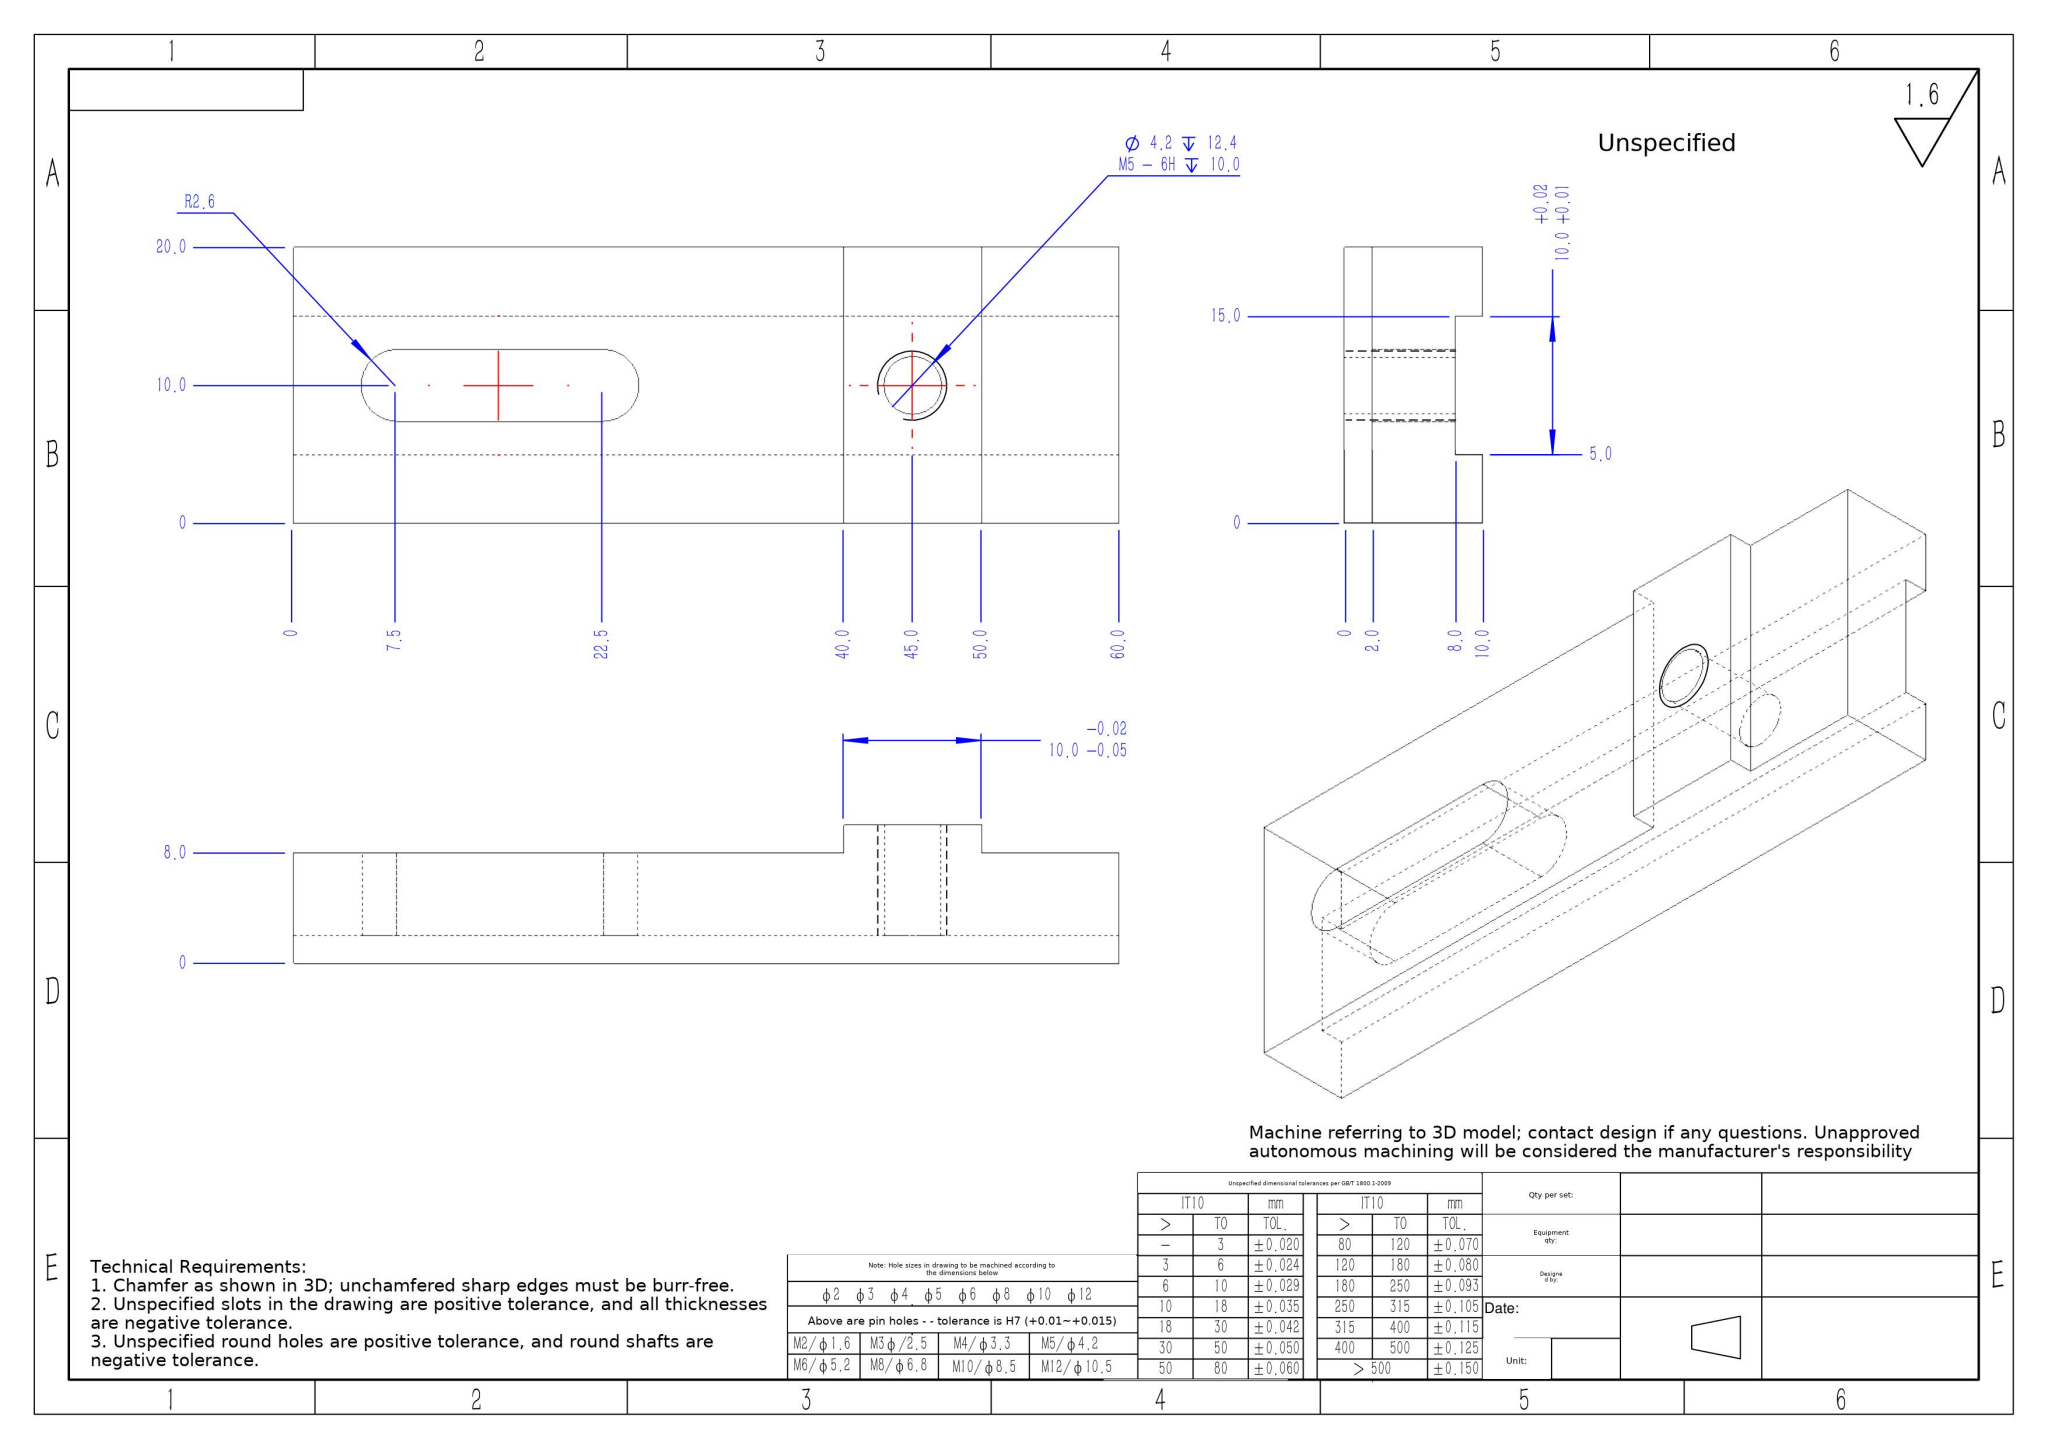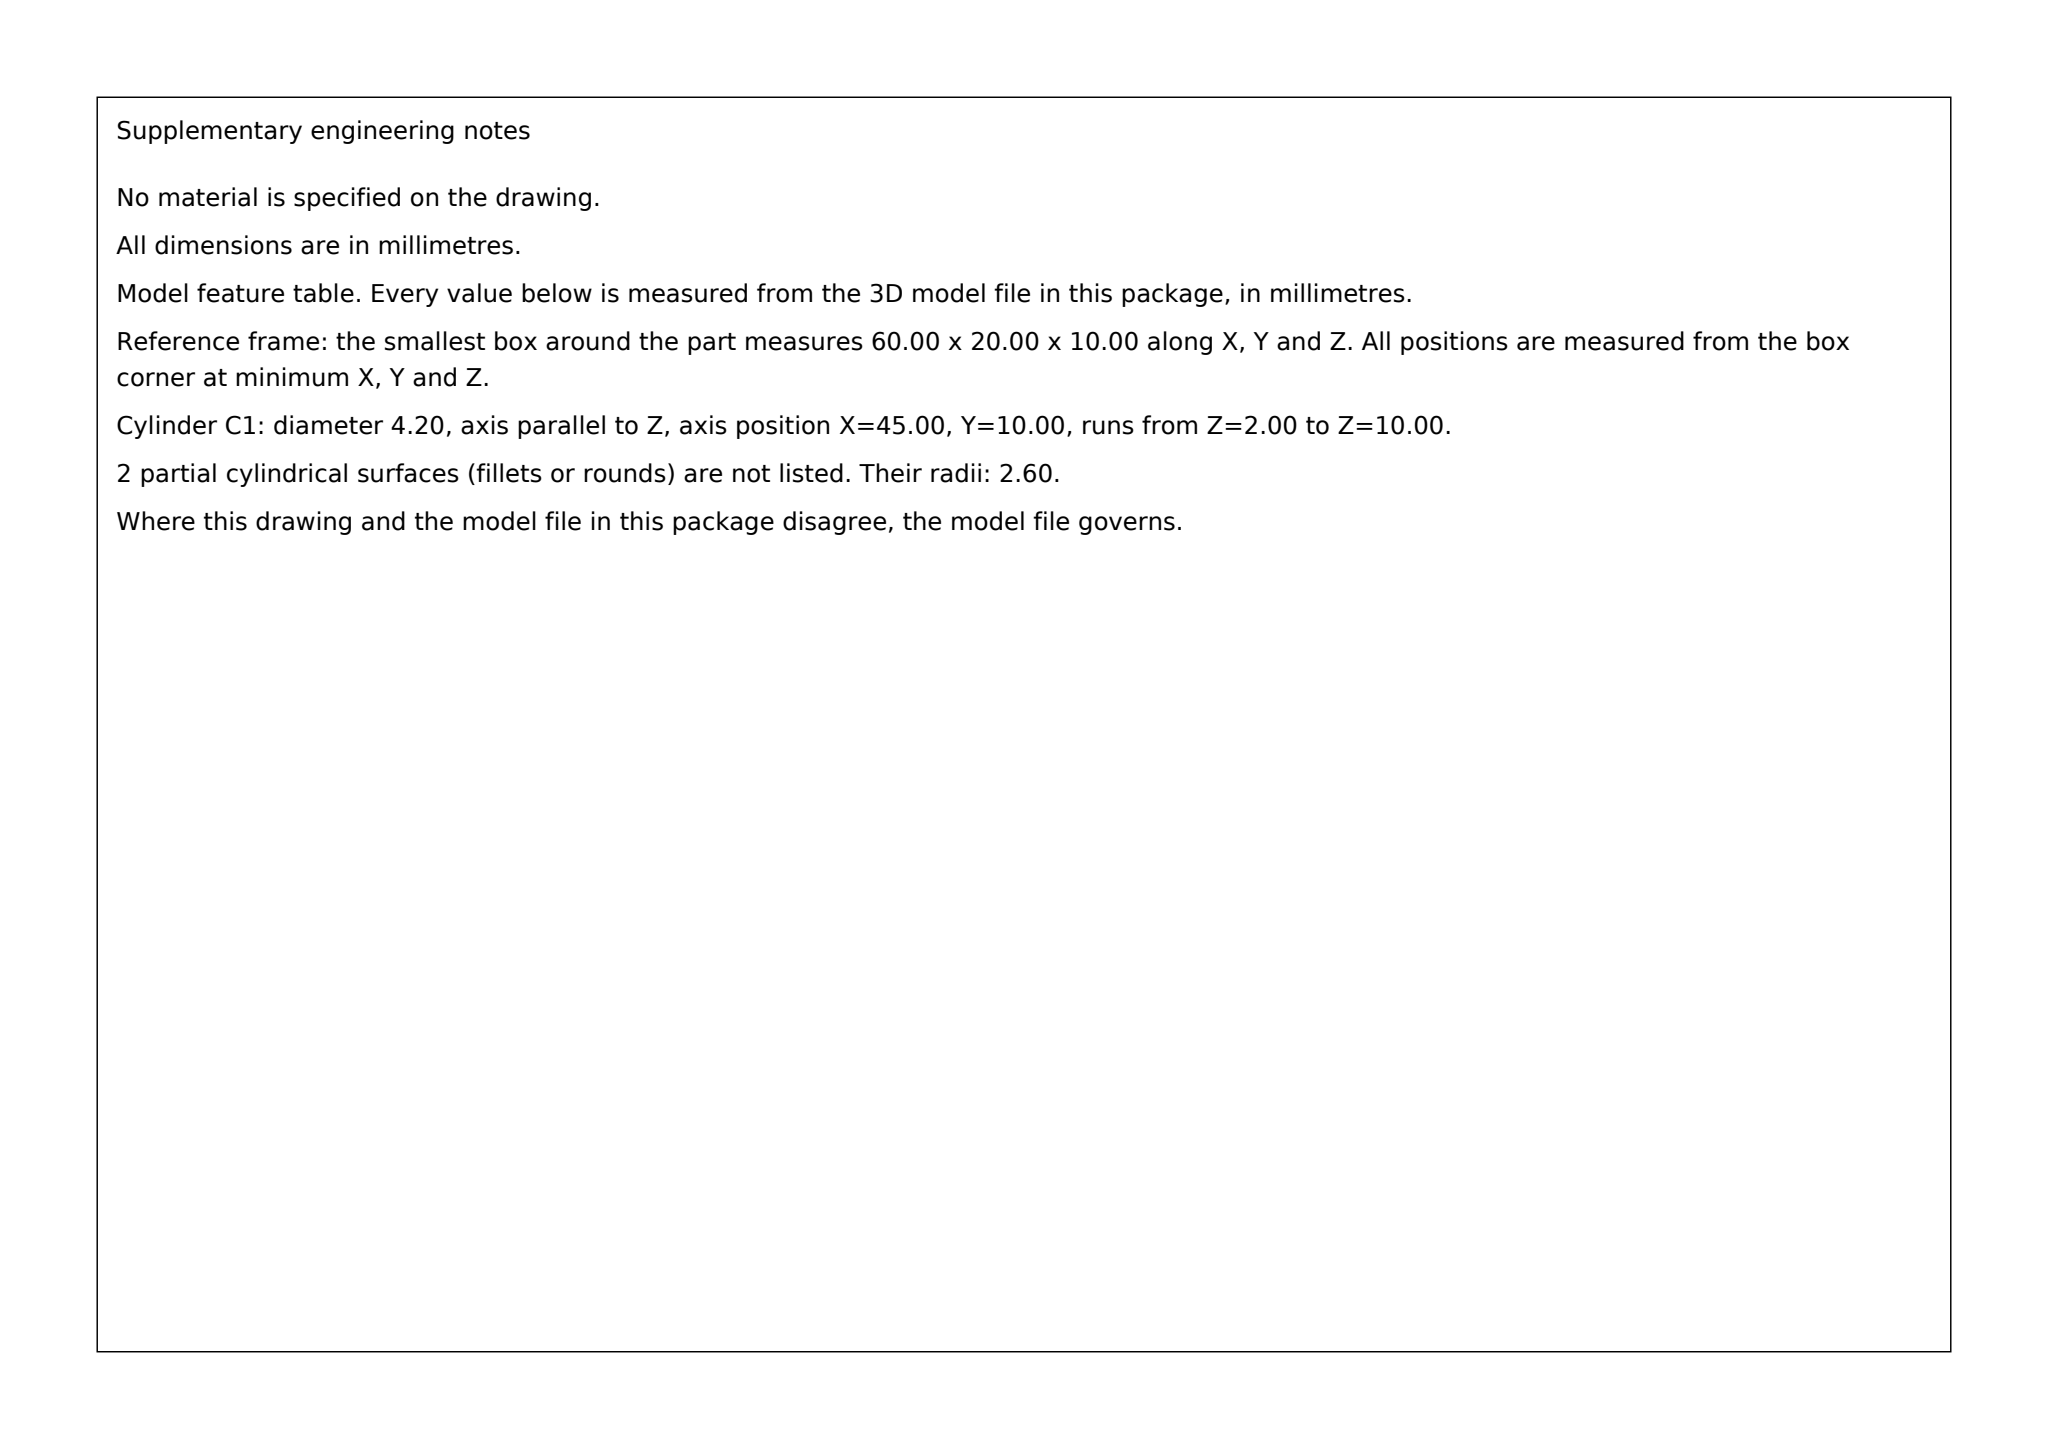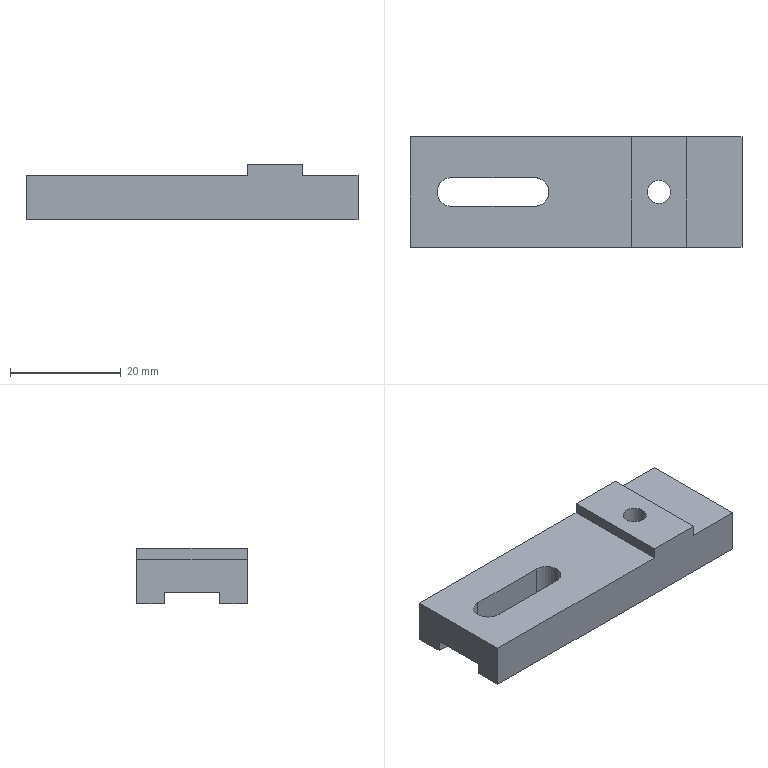Part | SolidWorks | mm | 1 solid | 21 faces | box 60 x 20 x 10 mm | volume 8094 mm3 | plane 16 | cylinder 5 | commonest cylinder face diameters 5.2 x3 4.2 x2
build123d program:
from build123d import *

# Parameters (mm, degrees)
SKETCH1_W             = 60
SKETCH1_H             = 20
BOSS_EXTRUDE1_DEPTH   = 4
SKETCH2_W             = 60
SKETCH2_H             = 10
CUT_EXTRUDE1_DEPTH    = 2
SKETCH3_W             = 10
SKETCH3_H             = 20
BOSS_EXTRUDE2_DEPTH   = 2
M5_TAPPED_HOLE1_D     = 4.2
M5_TAPPED_HOLE1_DEPTH = 12.4
M5_TAPPED_HOLE1_TIP   = 1.262
CUT_EXTRUDE2_DEPTH    = 39


with BuildPart() as part:
    # Sketch1 → Boss-Extrude1 (new, symmetric)
    with BuildSketch(Plane.XY):
        Rectangle(SKETCH1_W, SKETCH1_H)
    extrude(amount=BOSS_EXTRUDE1_DEPTH, both=True)

    # Sketch2 → Cut-Extrude1 (cut)
    with BuildSketch(Plane(origin=(0, 0, -4), x_dir=(-1, 0, 0), z_dir=(0, 0, -1))):
        Rectangle(SKETCH2_W, SKETCH2_H)
    extrude(amount=-CUT_EXTRUDE1_DEPTH, mode=Mode.SUBTRACT)

    # Sketch3 → Boss-Extrude2 (add)
    with BuildSketch(Plane.XY.offset(4)):
        with Locations((15, 0)):
            Rectangle(SKETCH3_W, SKETCH3_H)
    extrude(amount=BOSS_EXTRUDE2_DEPTH)

    # M5 Tapped Hole1
    with Locations(Plane.XY.offset(6)):
        with Locations((15, 0)):
            Hole(M5_TAPPED_HOLE1_D / 2, depth=M5_TAPPED_HOLE1_DEPTH)
            with Locations((0, 0, -(M5_TAPPED_HOLE1_DEPTH + M5_TAPPED_HOLE1_TIP / 2))):  # 118° drill point
                Cone(0, M5_TAPPED_HOLE1_D / 2, M5_TAPPED_HOLE1_TIP, mode=Mode.SUBTRACT)

    # Sketch6 → Cut-Extrude2 (cut)
    with BuildSketch(Plane.XY.offset(4)):
        with BuildLine():
            Line((-22.5, 2.6), (-7.5, 2.6))
            ThreePointArc((-7.5, 2.6), (-4.9, 0), (-7.5, -2.6))
            Line((-7.5, -2.6), (-22.5, -2.6))
            ThreePointArc((-22.5, -2.6), (-25.1, 0), (-22.5, 2.6))
        make_face()
    extrude(amount=-CUT_EXTRUDE2_DEPTH, mode=Mode.SUBTRACT)


solid = part.part